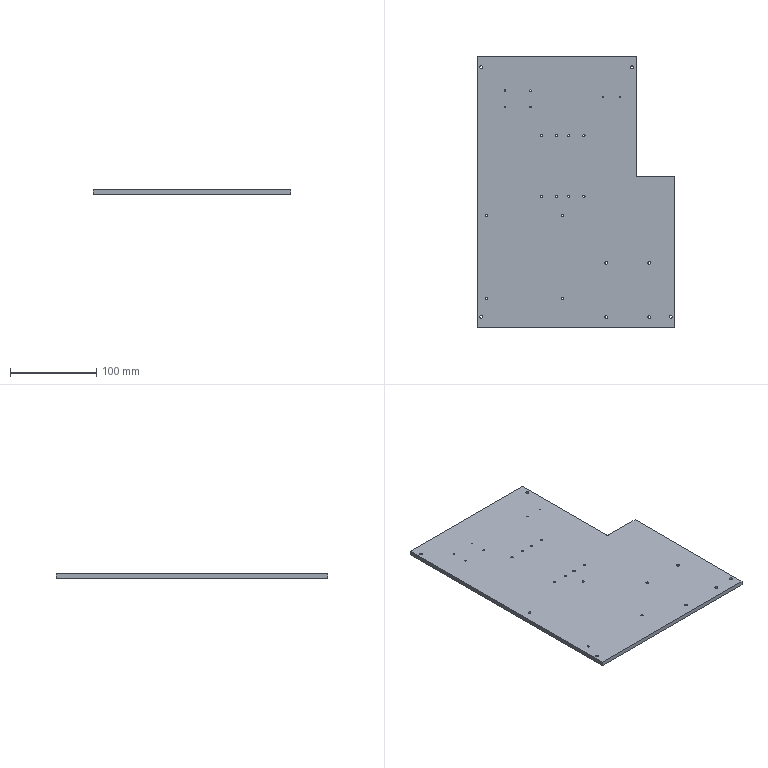CAM job | Mastercam | mm | 6 operations | part box 230 x 315.9 x 5
1. Contour (Ramp) | 10 - 10 平铣刀
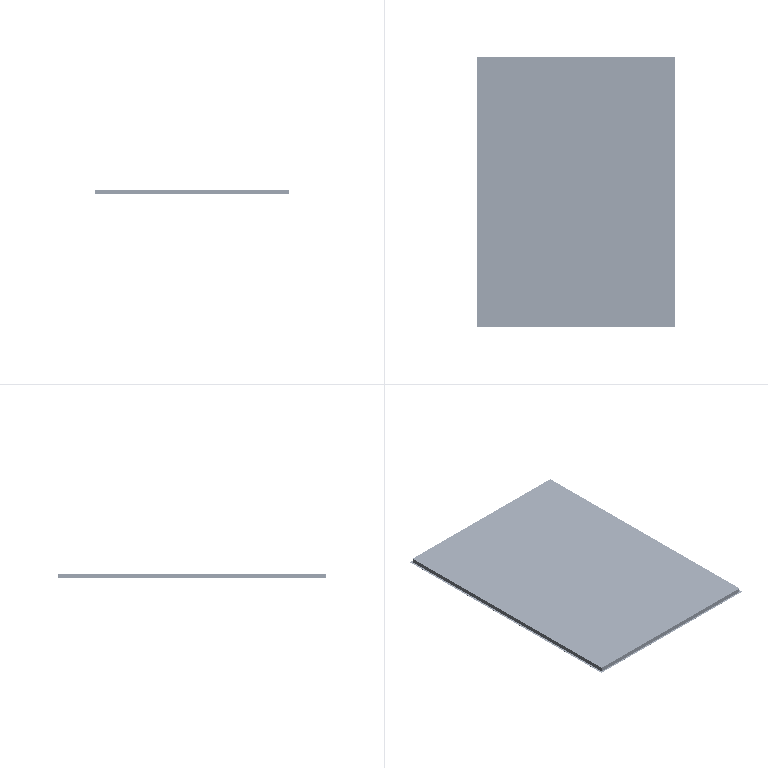2. Contour (2D) | 10 - 10 平铣刀
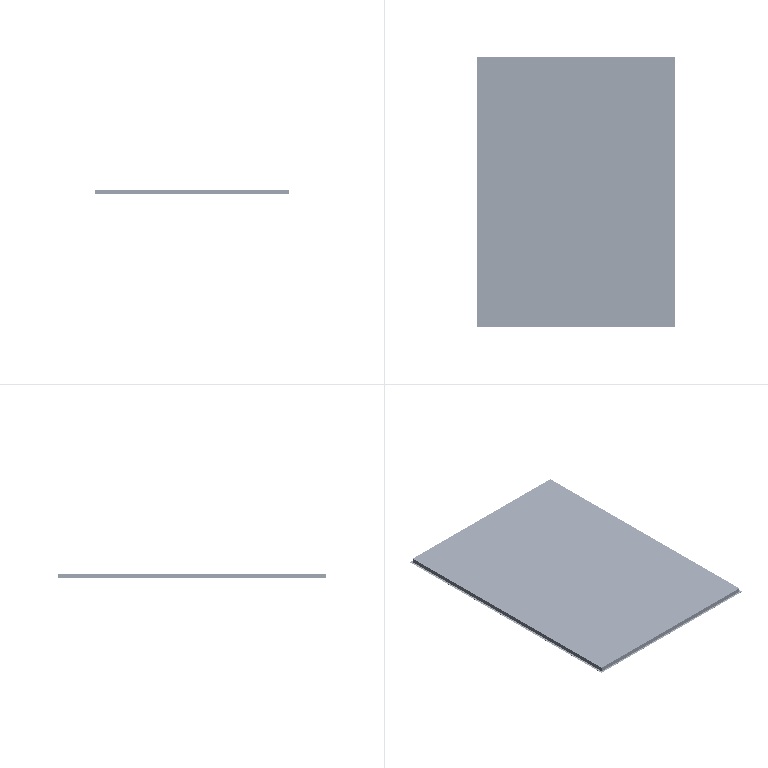3. Contour (Ramp) | 3 - 3 平铣刀
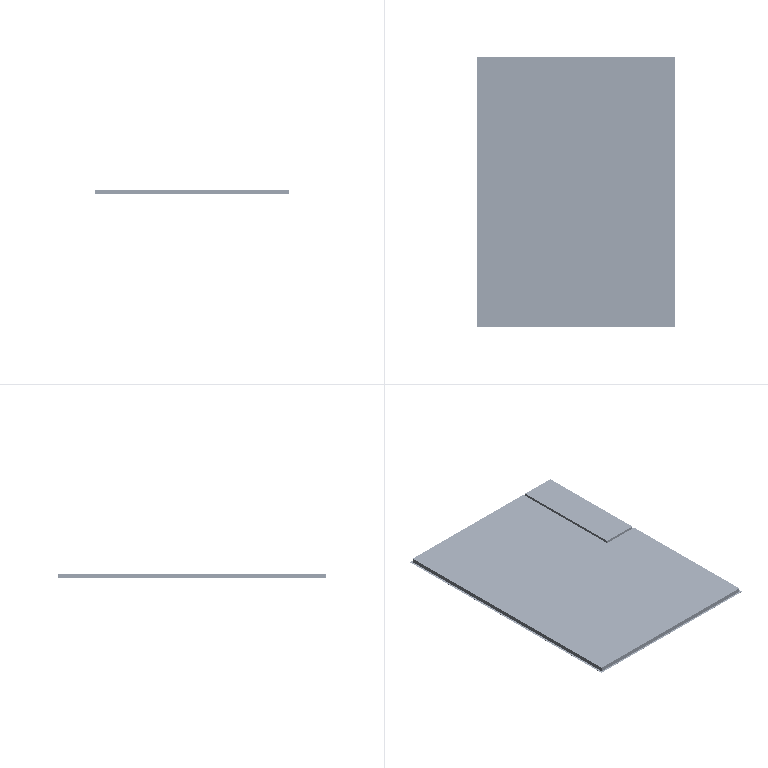4. Contour (2D) | 3 - 3 平铣刀
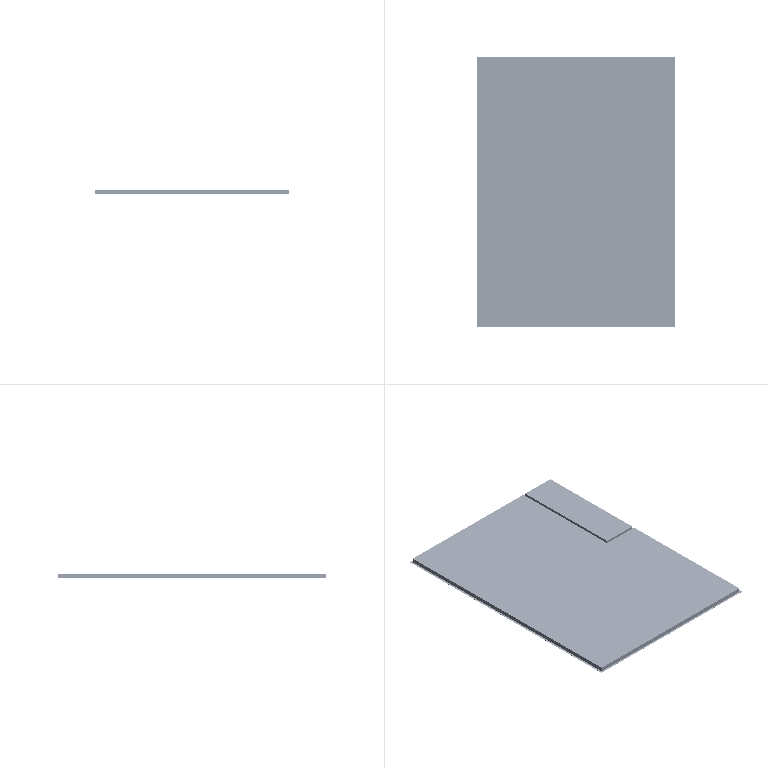5. Drill/Counterbore | 7 - 4 倒角刀
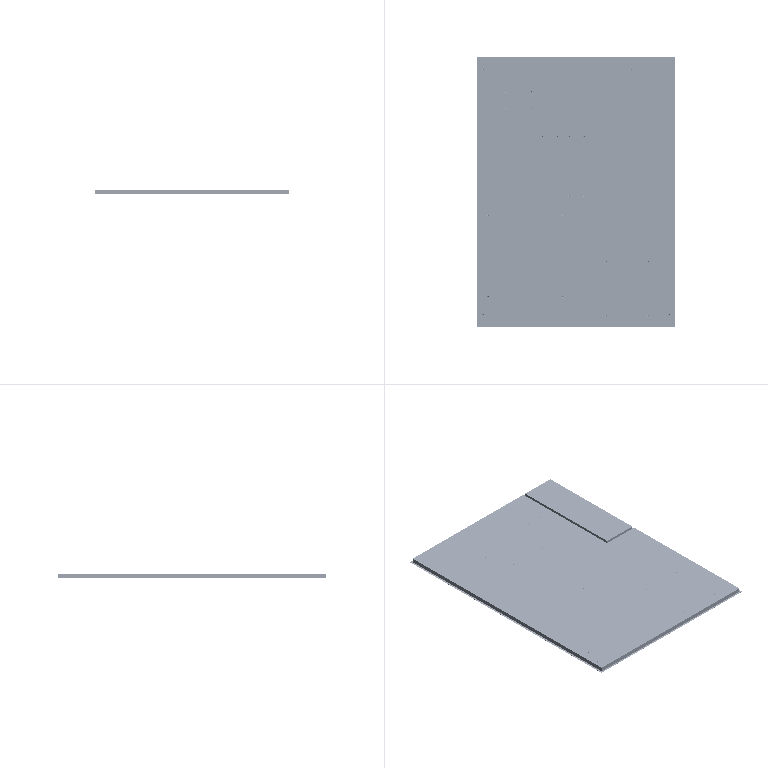6. Contour (2D chamfer) | 7 - 4 倒角刀